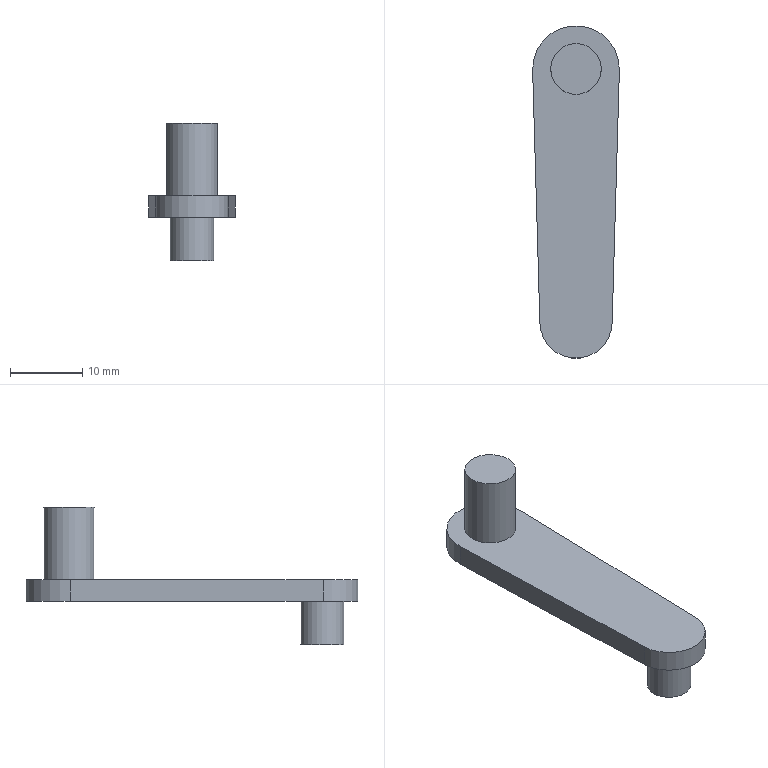Component | NX | CON_ROD5_2 | 1 solid | 10 faces | box 12 x 46 x 19 mm | volume 1997 mm3 | plane 6 | cylinder 4 | commonest cylinder face diameters 12 x1 10 x1 6 x1 7 x1
STEP:
#1=CARTESIAN_POINT('',(0.,0.,0.));
#2=DIRECTION('',(0.,0.,1.));
#3=DIRECTION('',(1.,0.,0.));
#4=AXIS2_PLACEMENT_3D('',#1,#2,#3);
#5=CARTESIAN_POINT('',(4.998,64.857,36.));
#6=VERTEX_POINT('',#5);
#7=CARTESIAN_POINT('',(5.998,99.829,36.));
#8=VERTEX_POINT('',#7);
#9=CARTESIAN_POINT('',(4.998,64.857,36.));
#10=DIRECTION('',(0.02857,0.9996,0.));
#11=VECTOR('',#10,1.);
#12=LINE('',#9,#11);
#13=CARTESIAN_POINT('',(4.998,64.857,39.));
#14=DIRECTION('',(-0.9996,0.02857,0.));
#15=DIRECTION('',(-0.02857,-0.9996,0.));
#16=AXIS2_PLACEMENT_3D('',#13,#14,#15);
#17=PLANE('',#16);
#18=CARTESIAN_POINT('',(0.,-3.));
#19=DIRECTION('',(-1.,0.));
#20=VECTOR('',#19,1.);
#21=LINE('',#18,#20);
#22=(GEOMETRIC_REPRESENTATION_CONTEXT(2)PARAMETRIC_REPRESENTATION_CONTEXT()REPRESENTATION_CONTEXT('',''));
#23=DEFINITIONAL_REPRESENTATION('',(#21),#22);
#24=PCURVE('',#17,#23);
#25=CARTESIAN_POINT('',(-0.,100.,36.));
#26=DIRECTION('',(0.,0.,1.));
#27=DIRECTION('',(-1.,0.,0.));
#28=AXIS2_PLACEMENT_3D('',#25,#26,#27);
#29=PLANE('',#28);
#30=CARTESIAN_POINT('',(-4.998,35.143));
#31=DIRECTION('',(-0.02857,-0.9996));
#32=VECTOR('',#31,1.);
#33=LINE('',#30,#32);
#34=(GEOMETRIC_REPRESENTATION_CONTEXT(2)PARAMETRIC_REPRESENTATION_CONTEXT()REPRESENTATION_CONTEXT('',''));
#35=DEFINITIONAL_REPRESENTATION('',(#33),#34);
#36=PCURVE('',#29,#35);
#37=SURFACE_CURVE('',#12,(#24,#36),.PCURVE_S1.);
#38=EDGE_CURVE('',#6,#8,#37,.T.);
#39=ORIENTED_EDGE('',*,*,#38,.T.);
#40=CARTESIAN_POINT('',(5.998,99.829,39.));
#41=VERTEX_POINT('',#40);
#42=CARTESIAN_POINT('',(5.998,99.829,39.));
#43=DIRECTION('',(0.,0.,-1.));
#44=VECTOR('',#43,1.);
#45=LINE('',#42,#44);
#46=CARTESIAN_POINT('',(-34.986,0.));
#47=DIRECTION('',(0.,-1.));
#48=VECTOR('',#47,1.);
#49=LINE('',#46,#48);
#50=(GEOMETRIC_REPRESENTATION_CONTEXT(2)PARAMETRIC_REPRESENTATION_CONTEXT()REPRESENTATION_CONTEXT('',''));
#51=DEFINITIONAL_REPRESENTATION('',(#49),#50);
#52=PCURVE('',#17,#51);
#53=CARTESIAN_POINT('',(-0.,100.,39.));
#54=DIRECTION('',(0.,0.,-1.));
#55=DIRECTION('',(1.,0.,0.));
#56=AXIS2_PLACEMENT_3D('',#53,#54,#55);
#57=CYLINDRICAL_SURFACE('',#56,6.);
#58=CARTESIAN_POINT('',(6.312,0.));
#59=DIRECTION('',(0.,1.));
#60=VECTOR('',#59,1.);
#61=LINE('',#58,#60);
#62=(GEOMETRIC_REPRESENTATION_CONTEXT(2)PARAMETRIC_REPRESENTATION_CONTEXT()REPRESENTATION_CONTEXT('',''));
#63=DEFINITIONAL_REPRESENTATION('',(#61),#62);
#64=PCURVE('',#57,#63);
#65=SURFACE_CURVE('',#45,(#52,#64),.PCURVE_S1.);
#66=EDGE_CURVE('',#41,#8,#65,.T.);
#67=ORIENTED_EDGE('',*,*,#66,.F.);
#68=CARTESIAN_POINT('',(4.998,64.857,39.));
#69=VERTEX_POINT('',#68);
#70=CARTESIAN_POINT('',(4.998,64.857,39.));
#71=DIRECTION('',(0.02857,0.9996,0.));
#72=VECTOR('',#71,1.);
#73=LINE('',#70,#72);
#74=CARTESIAN_POINT('',(0.,0.));
#75=DIRECTION('',(-1.,0.));
#76=VECTOR('',#75,1.);
#77=LINE('',#74,#76);
#78=(GEOMETRIC_REPRESENTATION_CONTEXT(2)PARAMETRIC_REPRESENTATION_CONTEXT()REPRESENTATION_CONTEXT('',''));
#79=DEFINITIONAL_REPRESENTATION('',(#77),#78);
#80=PCURVE('',#17,#79);
#81=CARTESIAN_POINT('',(-0.,100.,39.));
#82=DIRECTION('',(0.,0.,1.));
#83=DIRECTION('',(-1.,0.,0.));
#84=AXIS2_PLACEMENT_3D('',#81,#82,#83);
#85=PLANE('',#84);
#86=CARTESIAN_POINT('',(-4.998,35.143));
#87=DIRECTION('',(-0.02857,-0.9996));
#88=VECTOR('',#87,1.);
#89=LINE('',#86,#88);
#90=(GEOMETRIC_REPRESENTATION_CONTEXT(2)PARAMETRIC_REPRESENTATION_CONTEXT()REPRESENTATION_CONTEXT('',''));
#91=DEFINITIONAL_REPRESENTATION('',(#89),#90);
#92=PCURVE('',#85,#91);
#93=SURFACE_CURVE('',#73,(#80,#92),.PCURVE_S1.);
#94=EDGE_CURVE('',#69,#41,#93,.T.);
#95=ORIENTED_EDGE('',*,*,#94,.F.);
#96=CARTESIAN_POINT('',(4.998,64.857,39.));
#97=DIRECTION('',(0.,0.,-1.));
#98=VECTOR('',#97,1.);
#99=LINE('',#96,#98);
#100=CARTESIAN_POINT('',(0.,0.));
#101=DIRECTION('',(0.,-1.));
#102=VECTOR('',#101,1.);
#103=LINE('',#100,#102);
#104=(GEOMETRIC_REPRESENTATION_CONTEXT(2)PARAMETRIC_REPRESENTATION_CONTEXT()REPRESENTATION_CONTEXT('',''));
#105=DEFINITIONAL_REPRESENTATION('',(#103),#104);
#106=PCURVE('',#17,#105);
#107=CARTESIAN_POINT('',(-0.,65.,39.));
#108=DIRECTION('',(0.,0.,-1.));
#109=DIRECTION('',(1.,0.,0.));
#110=AXIS2_PLACEMENT_3D('',#107,#108,#109);
#111=CYLINDRICAL_SURFACE('',#110,5.);
#112=CARTESIAN_POINT('',(0.02858,0.));
#113=DIRECTION('',(0.,1.));
#114=VECTOR('',#113,1.);
#115=LINE('',#112,#114);
#116=(GEOMETRIC_REPRESENTATION_CONTEXT(2)PARAMETRIC_REPRESENTATION_CONTEXT()REPRESENTATION_CONTEXT('',''));
#117=DEFINITIONAL_REPRESENTATION('',(#115),#116);
#118=PCURVE('',#111,#117);
#119=SURFACE_CURVE('',#99,(#106,#118),.PCURVE_S1.);
#120=EDGE_CURVE('',#69,#6,#119,.T.);
#121=ORIENTED_EDGE('',*,*,#120,.T.);
#122=EDGE_LOOP('',(#39,#67,#95,#121));
#123=FACE_BOUND('',#122,.T.);
#124=ADVANCED_FACE('',(#123),#17,.F.);
#125=CARTESIAN_POINT('',(-5.998,99.829,36.));
#126=VERTEX_POINT('',#125);
#127=CARTESIAN_POINT('',(-0.,100.,36.));
#128=DIRECTION('',(0.,0.,1.));
#129=DIRECTION('',(-1.,0.,0.));
#130=AXIS2_PLACEMENT_3D('',#127,#128,#129);
#131=CIRCLE('',#130,6.);
#132=CARTESIAN_POINT('',(9.425,3.));
#133=DIRECTION('',(-1.,0.));
#134=VECTOR('',#133,1.);
#135=LINE('',#132,#134);
#136=(GEOMETRIC_REPRESENTATION_CONTEXT(2)PARAMETRIC_REPRESENTATION_CONTEXT()REPRESENTATION_CONTEXT('',''));
#137=DEFINITIONAL_REPRESENTATION('',(#135),#136);
#138=PCURVE('',#57,#137);
#139=CARTESIAN_POINT('',(0.,0.));
#140=DIRECTION('',(1.,0.));
#141=AXIS2_PLACEMENT_2D('',#139,#140);
#142=CIRCLE('',#141,6.);
#143=(GEOMETRIC_REPRESENTATION_CONTEXT(2)PARAMETRIC_REPRESENTATION_CONTEXT()REPRESENTATION_CONTEXT('',''));
#144=DEFINITIONAL_REPRESENTATION('',(#142),#143);
#145=PCURVE('',#29,#144);
#146=SURFACE_CURVE('',#131,(#138,#145),.PCURVE_S1.);
#147=EDGE_CURVE('',#8,#126,#146,.T.);
#148=ORIENTED_EDGE('',*,*,#147,.T.);
#149=CARTESIAN_POINT('',(-5.998,99.829,39.));
#150=VERTEX_POINT('',#149);
#151=CARTESIAN_POINT('',(-5.998,99.829,39.));
#152=DIRECTION('',(0.,0.,-1.));
#153=VECTOR('',#152,1.);
#154=LINE('',#151,#153);
#155=CARTESIAN_POINT('',(3.113,0.));
#156=DIRECTION('',(0.,1.));
#157=VECTOR('',#156,1.);
#158=LINE('',#155,#157);
#159=(GEOMETRIC_REPRESENTATION_CONTEXT(2)PARAMETRIC_REPRESENTATION_CONTEXT()REPRESENTATION_CONTEXT('',''));
#160=DEFINITIONAL_REPRESENTATION('',(#158),#159);
#161=PCURVE('',#57,#160);
#162=CARTESIAN_POINT('',(-5.998,99.829,39.));
#163=DIRECTION('',(0.9996,0.02857,0.));
#164=DIRECTION('',(-0.02857,0.9996,0.));
#165=AXIS2_PLACEMENT_3D('',#162,#163,#164);
#166=PLANE('',#165);
#167=CARTESIAN_POINT('',(0.,0.));
#168=DIRECTION('',(0.,-1.));
#169=VECTOR('',#168,1.);
#170=LINE('',#167,#169);
#171=(GEOMETRIC_REPRESENTATION_CONTEXT(2)PARAMETRIC_REPRESENTATION_CONTEXT()REPRESENTATION_CONTEXT('',''));
#172=DEFINITIONAL_REPRESENTATION('',(#170),#171);
#173=PCURVE('',#166,#172);
#174=SURFACE_CURVE('',#154,(#161,#173),.PCURVE_S1.);
#175=EDGE_CURVE('',#150,#126,#174,.T.);
#176=ORIENTED_EDGE('',*,*,#175,.F.);
#177=CARTESIAN_POINT('',(-0.,100.,39.));
#178=DIRECTION('',(0.,0.,1.));
#179=DIRECTION('',(-1.,0.,0.));
#180=AXIS2_PLACEMENT_3D('',#177,#178,#179);
#181=CIRCLE('',#180,6.);
#182=CARTESIAN_POINT('',(9.425,0.));
#183=DIRECTION('',(-1.,0.));
#184=VECTOR('',#183,1.);
#185=LINE('',#182,#184);
#186=(GEOMETRIC_REPRESENTATION_CONTEXT(2)PARAMETRIC_REPRESENTATION_CONTEXT()REPRESENTATION_CONTEXT('',''));
#187=DEFINITIONAL_REPRESENTATION('',(#185),#186);
#188=PCURVE('',#57,#187);
#189=CARTESIAN_POINT('',(0.,0.));
#190=DIRECTION('',(1.,0.));
#191=AXIS2_PLACEMENT_2D('',#189,#190);
#192=CIRCLE('',#191,6.);
#193=(GEOMETRIC_REPRESENTATION_CONTEXT(2)PARAMETRIC_REPRESENTATION_CONTEXT()REPRESENTATION_CONTEXT('',''));
#194=DEFINITIONAL_REPRESENTATION('',(#192),#193);
#195=PCURVE('',#85,#194);
#196=SURFACE_CURVE('',#181,(#188,#195),.PCURVE_S1.);
#197=EDGE_CURVE('',#41,#150,#196,.T.);
#198=ORIENTED_EDGE('',*,*,#197,.F.);
#199=ORIENTED_EDGE('',*,*,#66,.T.);
#200=EDGE_LOOP('',(#148,#176,#198,#199));
#201=FACE_BOUND('',#200,.T.);
#202=ADVANCED_FACE('',(#201),#57,.T.);
#203=CARTESIAN_POINT('',(-4.998,64.857,36.));
#204=VERTEX_POINT('',#203);
#205=CARTESIAN_POINT('',(-5.998,99.829,36.));
#206=DIRECTION('',(0.02857,-0.9996,0.));
#207=VECTOR('',#206,1.);
#208=LINE('',#205,#207);
#209=CARTESIAN_POINT('',(0.,-3.));
#210=DIRECTION('',(-1.,0.));
#211=VECTOR('',#210,1.);
#212=LINE('',#209,#211);
#213=(GEOMETRIC_REPRESENTATION_CONTEXT(2)PARAMETRIC_REPRESENTATION_CONTEXT()REPRESENTATION_CONTEXT('',''));
#214=DEFINITIONAL_REPRESENTATION('',(#212),#213);
#215=PCURVE('',#166,#214);
#216=CARTESIAN_POINT('',(5.998,0.1714));
#217=DIRECTION('',(-0.02857,0.9996));
#218=VECTOR('',#217,1.);
#219=LINE('',#216,#218);
#220=(GEOMETRIC_REPRESENTATION_CONTEXT(2)PARAMETRIC_REPRESENTATION_CONTEXT()REPRESENTATION_CONTEXT('',''));
#221=DEFINITIONAL_REPRESENTATION('',(#219),#220);
#222=PCURVE('',#29,#221);
#223=SURFACE_CURVE('',#208,(#215,#222),.PCURVE_S1.);
#224=EDGE_CURVE('',#126,#204,#223,.T.);
#225=ORIENTED_EDGE('',*,*,#224,.T.);
#226=CARTESIAN_POINT('',(-4.998,64.857,39.));
#227=VERTEX_POINT('',#226);
#228=CARTESIAN_POINT('',(-4.998,64.857,39.));
#229=DIRECTION('',(0.,0.,-1.));
#230=VECTOR('',#229,1.);
#231=LINE('',#228,#230);
#232=CARTESIAN_POINT('',(-34.986,0.));
#233=DIRECTION('',(0.,-1.));
#234=VECTOR('',#233,1.);
#235=LINE('',#232,#234);
#236=(GEOMETRIC_REPRESENTATION_CONTEXT(2)PARAMETRIC_REPRESENTATION_CONTEXT()REPRESENTATION_CONTEXT('',''));
#237=DEFINITIONAL_REPRESENTATION('',(#235),#236);
#238=PCURVE('',#166,#237);
#239=CARTESIAN_POINT('',(3.113,0.));
#240=DIRECTION('',(0.,1.));
#241=VECTOR('',#240,1.);
#242=LINE('',#239,#241);
#243=(GEOMETRIC_REPRESENTATION_CONTEXT(2)PARAMETRIC_REPRESENTATION_CONTEXT()REPRESENTATION_CONTEXT('',''));
#244=DEFINITIONAL_REPRESENTATION('',(#242),#243);
#245=PCURVE('',#111,#244);
#246=SURFACE_CURVE('',#231,(#238,#245),.PCURVE_S1.);
#247=EDGE_CURVE('',#227,#204,#246,.T.);
#248=ORIENTED_EDGE('',*,*,#247,.F.);
#249=CARTESIAN_POINT('',(-5.998,99.829,39.));
#250=DIRECTION('',(0.02857,-0.9996,0.));
#251=VECTOR('',#250,1.);
#252=LINE('',#249,#251);
#253=CARTESIAN_POINT('',(0.,0.));
#254=DIRECTION('',(-1.,0.));
#255=VECTOR('',#254,1.);
#256=LINE('',#253,#255);
#257=(GEOMETRIC_REPRESENTATION_CONTEXT(2)PARAMETRIC_REPRESENTATION_CONTEXT()REPRESENTATION_CONTEXT('',''));
#258=DEFINITIONAL_REPRESENTATION('',(#256),#257);
#259=PCURVE('',#166,#258);
#260=CARTESIAN_POINT('',(5.998,0.1714));
#261=DIRECTION('',(-0.02857,0.9996));
#262=VECTOR('',#261,1.);
#263=LINE('',#260,#262);
#264=(GEOMETRIC_REPRESENTATION_CONTEXT(2)PARAMETRIC_REPRESENTATION_CONTEXT()REPRESENTATION_CONTEXT('',''));
#265=DEFINITIONAL_REPRESENTATION('',(#263),#264);
#266=PCURVE('',#85,#265);
#267=SURFACE_CURVE('',#252,(#259,#266),.PCURVE_S1.);
#268=EDGE_CURVE('',#150,#227,#267,.T.);
#269=ORIENTED_EDGE('',*,*,#268,.F.);
#270=ORIENTED_EDGE('',*,*,#175,.T.);
#271=EDGE_LOOP('',(#225,#248,#269,#270));
#272=FACE_BOUND('',#271,.T.);
#273=ADVANCED_FACE('',(#272),#166,.F.);
#274=CARTESIAN_POINT('',(-0.,65.,36.));
#275=DIRECTION('',(0.,0.,1.));
#276=DIRECTION('',(-1.,0.,0.));
#277=AXIS2_PLACEMENT_3D('',#274,#275,#276);
#278=CIRCLE('',#277,5.);
#279=CARTESIAN_POINT('',(3.142,3.));
#280=DIRECTION('',(-1.,0.));
#281=VECTOR('',#280,1.);
#282=LINE('',#279,#281);
#283=(GEOMETRIC_REPRESENTATION_CONTEXT(2)PARAMETRIC_REPRESENTATION_CONTEXT()REPRESENTATION_CONTEXT('',''));
#284=DEFINITIONAL_REPRESENTATION('',(#282),#283);
#285=PCURVE('',#111,#284);
#286=CARTESIAN_POINT('',(0.,35.));
#287=DIRECTION('',(1.,0.));
#288=AXIS2_PLACEMENT_2D('',#286,#287);
#289=CIRCLE('',#288,5.);
#290=(GEOMETRIC_REPRESENTATION_CONTEXT(2)PARAMETRIC_REPRESENTATION_CONTEXT()REPRESENTATION_CONTEXT('',''));
#291=DEFINITIONAL_REPRESENTATION('',(#289),#290);
#292=PCURVE('',#29,#291);
#293=SURFACE_CURVE('',#278,(#285,#292),.PCURVE_S1.);
#294=EDGE_CURVE('',#204,#6,#293,.T.);
#295=ORIENTED_EDGE('',*,*,#294,.T.);
#296=ORIENTED_EDGE('',*,*,#120,.F.);
#297=CARTESIAN_POINT('',(-0.,65.,39.));
#298=DIRECTION('',(0.,0.,1.));
#299=DIRECTION('',(-1.,0.,0.));
#300=AXIS2_PLACEMENT_3D('',#297,#298,#299);
#301=CIRCLE('',#300,5.);
#302=CARTESIAN_POINT('',(3.142,0.));
#303=DIRECTION('',(-1.,0.));
#304=VECTOR('',#303,1.);
#305=LINE('',#302,#304);
#306=(GEOMETRIC_REPRESENTATION_CONTEXT(2)PARAMETRIC_REPRESENTATION_CONTEXT()REPRESENTATION_CONTEXT('',''));
#307=DEFINITIONAL_REPRESENTATION('',(#305),#306);
#308=PCURVE('',#111,#307);
#309=CARTESIAN_POINT('',(0.,35.));
#310=DIRECTION('',(1.,0.));
#311=AXIS2_PLACEMENT_2D('',#309,#310);
#312=CIRCLE('',#311,5.);
#313=(GEOMETRIC_REPRESENTATION_CONTEXT(2)PARAMETRIC_REPRESENTATION_CONTEXT()REPRESENTATION_CONTEXT('',''));
#314=DEFINITIONAL_REPRESENTATION('',(#312),#313);
#315=PCURVE('',#85,#314);
#316=SURFACE_CURVE('',#301,(#308,#315),.PCURVE_S1.);
#317=EDGE_CURVE('',#227,#69,#316,.T.);
#318=ORIENTED_EDGE('',*,*,#317,.F.);
#319=ORIENTED_EDGE('',*,*,#247,.T.);
#320=EDGE_LOOP('',(#295,#296,#318,#319));
#321=FACE_BOUND('',#320,.T.);
#322=ADVANCED_FACE('',(#321),#111,.T.);
#323=CARTESIAN_POINT('',(-3.5,100.,39.));
#324=VERTEX_POINT('',#323);
#325=CARTESIAN_POINT('',(-0.,100.,39.));
#326=DIRECTION('',(0.,0.,1.));
#327=DIRECTION('',(-1.,0.,0.));
#328=AXIS2_PLACEMENT_3D('',#325,#326,#327);
#329=CIRCLE('',#328,3.5);
#330=CARTESIAN_POINT('',(0.,0.));
#331=DIRECTION('',(1.,0.));
#332=AXIS2_PLACEMENT_2D('',#330,#331);
#333=CIRCLE('',#332,3.5);
#334=(GEOMETRIC_REPRESENTATION_CONTEXT(2)PARAMETRIC_REPRESENTATION_CONTEXT()REPRESENTATION_CONTEXT('',''));
#335=DEFINITIONAL_REPRESENTATION('',(#333),#334);
#336=PCURVE('',#85,#335);
#337=CARTESIAN_POINT('',(-0.,100.,39.));
#338=DIRECTION('',(0.,0.,1.));
#339=DIRECTION('',(-1.,0.,0.));
#340=AXIS2_PLACEMENT_3D('',#337,#338,#339);
#341=CYLINDRICAL_SURFACE('',#340,3.5);
#342=CARTESIAN_POINT('',(0.,0.));
#343=DIRECTION('',(1.,0.));
#344=VECTOR('',#343,1.);
#345=LINE('',#342,#344);
#346=(GEOMETRIC_REPRESENTATION_CONTEXT(2)PARAMETRIC_REPRESENTATION_CONTEXT()REPRESENTATION_CONTEXT('',''));
#347=DEFINITIONAL_REPRESENTATION('',(#345),#346);
#348=PCURVE('',#341,#347);
#349=SURFACE_CURVE('',#329,(#336,#348),.PCURVE_S1.);
#350=EDGE_CURVE('',#324,#324,#349,.T.);
#351=ORIENTED_EDGE('',*,*,#350,.F.);
#352=EDGE_LOOP('',(#351));
#353=FACE_BOUND('',#352,.T.);
#354=ORIENTED_EDGE('',*,*,#94,.T.);
#355=ORIENTED_EDGE('',*,*,#197,.T.);
#356=ORIENTED_EDGE('',*,*,#268,.T.);
#357=ORIENTED_EDGE('',*,*,#317,.T.);
#358=EDGE_LOOP('',(#354,#355,#356,#357));
#359=FACE_BOUND('',#358,.T.);
#360=ADVANCED_FACE('',(#353,#359),#85,.T.);
#361=CARTESIAN_POINT('',(-3.,65.,36.));
#362=VERTEX_POINT('',#361);
#363=CARTESIAN_POINT('',(-0.,65.,36.));
#364=DIRECTION('',(0.,0.,-1.));
#365=DIRECTION('',(-1.,0.,0.));
#366=AXIS2_PLACEMENT_3D('',#363,#364,#365);
#367=CIRCLE('',#366,3.);
#368=CARTESIAN_POINT('',(3.,35.));
#369=CARTESIAN_POINT('',(3.,29.804));
#370=CARTESIAN_POINT('',(-1.5,32.402));
#371=CARTESIAN_POINT('',(-6.,35.));
#372=CARTESIAN_POINT('',(-1.5,37.598));
#373=CARTESIAN_POINT('',(3.,40.196));
#374=CARTESIAN_POINT('',(3.,35.));
#375=(BOUNDED_CURVE()B_SPLINE_CURVE(2,(#368,#369,#370,#371,#372,#373,#374),.UNSPECIFIED.,.T.,.F.)B_SPLINE_CURVE_WITH_KNOTS((1,2,2,2,2,1),(-2.094,0.,2.094,4.189,6.283,8.378),.UNSPECIFIED.)CURVE()GEOMETRIC_REPRESENTATION_ITEM()RATIONAL_B_SPLINE_CURVE((1.,0.5,1.,0.5,1.,0.5,1.))REPRESENTATION_ITEM(''));
#376=(GEOMETRIC_REPRESENTATION_CONTEXT(2)PARAMETRIC_REPRESENTATION_CONTEXT()REPRESENTATION_CONTEXT('',''));
#377=DEFINITIONAL_REPRESENTATION('',(#375),#376);
#378=PCURVE('',#29,#377);
#379=CARTESIAN_POINT('',(-0.,65.,36.));
#380=DIRECTION('',(0.,0.,-1.));
#381=DIRECTION('',(-1.,0.,0.));
#382=AXIS2_PLACEMENT_3D('',#379,#380,#381);
#383=CYLINDRICAL_SURFACE('',#382,3.);
#384=CARTESIAN_POINT('',(0.,0.));
#385=DIRECTION('',(1.,0.));
#386=VECTOR('',#385,1.);
#387=LINE('',#384,#386);
#388=(GEOMETRIC_REPRESENTATION_CONTEXT(2)PARAMETRIC_REPRESENTATION_CONTEXT()REPRESENTATION_CONTEXT('',''));
#389=DEFINITIONAL_REPRESENTATION('',(#387),#388);
#390=PCURVE('',#383,#389);
#391=SURFACE_CURVE('',#367,(#378,#390),.PCURVE_S1.);
#392=EDGE_CURVE('',#362,#362,#391,.T.);
#393=ORIENTED_EDGE('',*,*,#392,.F.);
#394=EDGE_LOOP('',(#393));
#395=FACE_BOUND('',#394,.T.);
#396=ORIENTED_EDGE('',*,*,#38,.F.);
#397=ORIENTED_EDGE('',*,*,#294,.F.);
#398=ORIENTED_EDGE('',*,*,#224,.F.);
#399=ORIENTED_EDGE('',*,*,#147,.F.);
#400=EDGE_LOOP('',(#396,#397,#398,#399));
#401=FACE_BOUND('',#400,.T.);
#402=ADVANCED_FACE('',(#395,#401),#29,.F.);
#403=CARTESIAN_POINT('',(-3.,65.,30.));
#404=VERTEX_POINT('',#403);
#405=CARTESIAN_POINT('',(-0.,65.,30.));
#406=DIRECTION('',(0.,0.,1.));
#407=DIRECTION('',(-1.,0.,0.));
#408=AXIS2_PLACEMENT_3D('',#405,#406,#407);
#409=CIRCLE('',#408,3.);
#410=CARTESIAN_POINT('',(-0.,65.,30.));
#411=DIRECTION('',(0.,0.,-1.));
#412=DIRECTION('',(1.,0.,0.));
#413=AXIS2_PLACEMENT_3D('',#410,#411,#412);
#414=PLANE('',#413);
#415=CARTESIAN_POINT('',(-3.,0.));
#416=CARTESIAN_POINT('',(-3.,5.196));
#417=CARTESIAN_POINT('',(1.5,2.598));
#418=CARTESIAN_POINT('',(6.,0.));
#419=CARTESIAN_POINT('',(1.5,-2.598));
#420=CARTESIAN_POINT('',(-3.,-5.196));
#421=CARTESIAN_POINT('',(-3.,0.));
#422=(BOUNDED_CURVE()B_SPLINE_CURVE(2,(#415,#416,#417,#418,#419,#420,#421),.UNSPECIFIED.,.T.,.F.)B_SPLINE_CURVE_WITH_KNOTS((1,2,2,2,2,1),(-2.094,0.,2.094,4.189,6.283,8.378),.UNSPECIFIED.)CURVE()GEOMETRIC_REPRESENTATION_ITEM()RATIONAL_B_SPLINE_CURVE((1.,0.5,1.,0.5,1.,0.5,1.))REPRESENTATION_ITEM(''));
#423=(GEOMETRIC_REPRESENTATION_CONTEXT(2)PARAMETRIC_REPRESENTATION_CONTEXT()REPRESENTATION_CONTEXT('',''));
#424=DEFINITIONAL_REPRESENTATION('',(#422),#423);
#425=PCURVE('',#414,#424);
#426=CARTESIAN_POINT('',(6.283,6.));
#427=DIRECTION('',(-1.,0.));
#428=VECTOR('',#427,1.);
#429=LINE('',#426,#428);
#430=(GEOMETRIC_REPRESENTATION_CONTEXT(2)PARAMETRIC_REPRESENTATION_CONTEXT()REPRESENTATION_CONTEXT('',''));
#431=DEFINITIONAL_REPRESENTATION('',(#429),#430);
#432=PCURVE('',#383,#431);
#433=SURFACE_CURVE('',#409,(#425,#432),.PCURVE_S1.);
#434=EDGE_CURVE('',#404,#404,#433,.T.);
#435=ORIENTED_EDGE('',*,*,#434,.F.);
#436=EDGE_LOOP('',(#435));
#437=FACE_BOUND('',#436,.T.);
#438=ADVANCED_FACE('',(#437),#414,.T.);
#439=ORIENTED_EDGE('',*,*,#434,.T.);
#440=CARTESIAN_POINT('',(-3.,65.,36.));
#441=CARTESIAN_POINT('',(-3.,65.,30.));
#442=B_SPLINE_CURVE_WITH_KNOTS('',1,(#440,#441),.UNSPECIFIED.,.F.,.F.,(2,2),(0.,6.),.PIECEWISE_BEZIER_KNOTS.);
#443=CARTESIAN_POINT('',(0.,0.));
#444=DIRECTION('',(0.,1.));
#445=VECTOR('',#444,1.);
#446=LINE('',#443,#445);
#447=(GEOMETRIC_REPRESENTATION_CONTEXT(2)PARAMETRIC_REPRESENTATION_CONTEXT()REPRESENTATION_CONTEXT('',''));
#448=DEFINITIONAL_REPRESENTATION('',(#446),#447);
#449=PCURVE('',#383,#448);
#450=CARTESIAN_POINT('',(6.283,0.));
#451=DIRECTION('',(0.,1.));
#452=VECTOR('',#451,1.);
#453=LINE('',#450,#452);
#454=(GEOMETRIC_REPRESENTATION_CONTEXT(2)PARAMETRIC_REPRESENTATION_CONTEXT()REPRESENTATION_CONTEXT('',''));
#455=DEFINITIONAL_REPRESENTATION('',(#453),#454);
#456=PCURVE('',#383,#455);
#457=SEAM_CURVE('',#442,(#449,#456),.PCURVE_S1.);
#458=EDGE_CURVE('',#362,#404,#457,.T.);
#459=ORIENTED_EDGE('',*,*,#458,.F.);
#460=ORIENTED_EDGE('',*,*,#392,.T.);
#461=ORIENTED_EDGE('',*,*,#458,.T.);
#462=EDGE_LOOP('',(#439,#459,#460,#461));
#463=FACE_BOUND('',#462,.T.);
#464=ADVANCED_FACE('',(#463),#383,.T.);
#465=CARTESIAN_POINT('',(-3.5,100.,49.));
#466=VERTEX_POINT('',#465);
#467=CARTESIAN_POINT('',(-0.,100.,49.));
#468=DIRECTION('',(0.,0.,-1.));
#469=DIRECTION('',(-1.,0.,0.));
#470=AXIS2_PLACEMENT_3D('',#467,#468,#469);
#471=CIRCLE('',#470,3.5);
#472=CARTESIAN_POINT('',(-0.,100.,49.));
#473=DIRECTION('',(0.,0.,1.));
#474=DIRECTION('',(-1.,0.,0.));
#475=AXIS2_PLACEMENT_3D('',#472,#473,#474);
#476=PLANE('',#475);
#477=CARTESIAN_POINT('',(3.5,0.));
#478=CARTESIAN_POINT('',(3.5,-6.062));
#479=CARTESIAN_POINT('',(-1.75,-3.031));
#480=CARTESIAN_POINT('',(-7.,-0.));
#481=CARTESIAN_POINT('',(-1.75,3.031));
#482=CARTESIAN_POINT('',(3.5,6.062));
#483=CARTESIAN_POINT('',(3.5,0.));
#484=(BOUNDED_CURVE()B_SPLINE_CURVE(2,(#477,#478,#479,#480,#481,#482,#483),.UNSPECIFIED.,.T.,.F.)B_SPLINE_CURVE_WITH_KNOTS((1,2,2,2,2,1),(-2.094,0.,2.094,4.189,6.283,8.378),.UNSPECIFIED.)CURVE()GEOMETRIC_REPRESENTATION_ITEM()RATIONAL_B_SPLINE_CURVE((1.,0.5,1.,0.5,1.,0.5,1.))REPRESENTATION_ITEM(''));
#485=(GEOMETRIC_REPRESENTATION_CONTEXT(2)PARAMETRIC_REPRESENTATION_CONTEXT()REPRESENTATION_CONTEXT('',''));
#486=DEFINITIONAL_REPRESENTATION('',(#484),#485);
#487=PCURVE('',#476,#486);
#488=CARTESIAN_POINT('',(6.283,10.));
#489=DIRECTION('',(-1.,0.));
#490=VECTOR('',#489,1.);
#491=LINE('',#488,#490);
#492=(GEOMETRIC_REPRESENTATION_CONTEXT(2)PARAMETRIC_REPRESENTATION_CONTEXT()REPRESENTATION_CONTEXT('',''));
#493=DEFINITIONAL_REPRESENTATION('',(#491),#492);
#494=PCURVE('',#341,#493);
#495=SURFACE_CURVE('',#471,(#487,#494),.PCURVE_S1.);
#496=EDGE_CURVE('',#466,#466,#495,.T.);
#497=ORIENTED_EDGE('',*,*,#496,.F.);
#498=EDGE_LOOP('',(#497));
#499=FACE_BOUND('',#498,.T.);
#500=ADVANCED_FACE('',(#499),#476,.T.);
#501=ORIENTED_EDGE('',*,*,#496,.T.);
#502=CARTESIAN_POINT('',(-3.5,100.,39.));
#503=CARTESIAN_POINT('',(-3.5,100.,49.));
#504=B_SPLINE_CURVE_WITH_KNOTS('',1,(#502,#503),.UNSPECIFIED.,.F.,.F.,(2,2),(0.,10.),.PIECEWISE_BEZIER_KNOTS.);
#505=CARTESIAN_POINT('',(0.,0.));
#506=DIRECTION('',(0.,1.));
#507=VECTOR('',#506,1.);
#508=LINE('',#505,#507);
#509=(GEOMETRIC_REPRESENTATION_CONTEXT(2)PARAMETRIC_REPRESENTATION_CONTEXT()REPRESENTATION_CONTEXT('',''));
#510=DEFINITIONAL_REPRESENTATION('',(#508),#509);
#511=PCURVE('',#341,#510);
#512=CARTESIAN_POINT('',(6.283,0.));
#513=DIRECTION('',(0.,1.));
#514=VECTOR('',#513,1.);
#515=LINE('',#512,#514);
#516=(GEOMETRIC_REPRESENTATION_CONTEXT(2)PARAMETRIC_REPRESENTATION_CONTEXT()REPRESENTATION_CONTEXT('',''));
#517=DEFINITIONAL_REPRESENTATION('',(#515),#516);
#518=PCURVE('',#341,#517);
#519=SEAM_CURVE('',#504,(#511,#518),.PCURVE_S1.);
#520=EDGE_CURVE('',#324,#466,#519,.T.);
#521=ORIENTED_EDGE('',*,*,#520,.F.);
#522=ORIENTED_EDGE('',*,*,#350,.T.);
#523=ORIENTED_EDGE('',*,*,#520,.T.);
#524=EDGE_LOOP('',(#501,#521,#522,#523));
#525=FACE_BOUND('',#524,.T.);
#526=ADVANCED_FACE('',(#525),#341,.T.);
#527=CLOSED_SHELL('',(#124,#202,#273,#322,#360,#402,#438,#464,#500,#526));
#528=MANIFOLD_SOLID_BREP('',#527);
#529=(LENGTH_UNIT()NAMED_UNIT(*)SI_UNIT(.MILLI.,.METRE.));
#530=UNCERTAINTY_MEASURE_WITH_UNIT(LENGTH_MEASURE(0.000002),#529,'','');
#531=(NAMED_UNIT(*)PLANE_ANGLE_UNIT()SI_UNIT($,.RADIAN.));
#532=(NAMED_UNIT(*)SI_UNIT($,.STERADIAN.)SOLID_ANGLE_UNIT());
#533=(GEOMETRIC_REPRESENTATION_CONTEXT(3)GLOBAL_UNCERTAINTY_ASSIGNED_CONTEXT((#530))GLOBAL_UNIT_ASSIGNED_CONTEXT((#529,#531,#532))REPRESENTATION_CONTEXT('',''));
#534=ADVANCED_BREP_SHAPE_REPRESENTATION('',(#4,#528),#533);